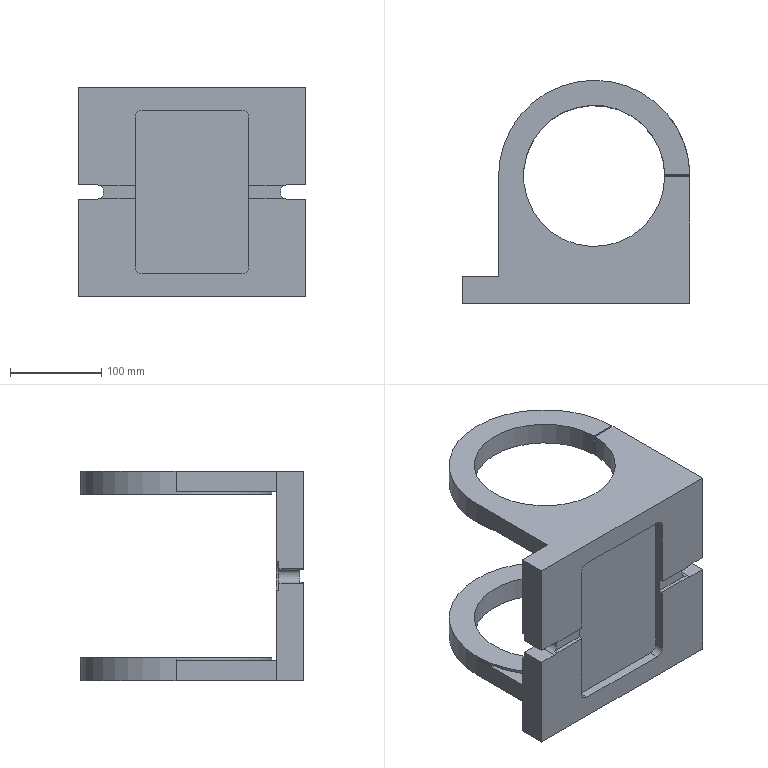Component | SolidWorks | 11Base-1 | 1 solid | 75 faces | volume 2365263 mm3 | plane 47 | cylinder 24 | cone 4 | commonest cylinder face diameters 16 x6 8.5 x4 11 x4 210 x3 32 x2 155 x2 17 x2 240 x1